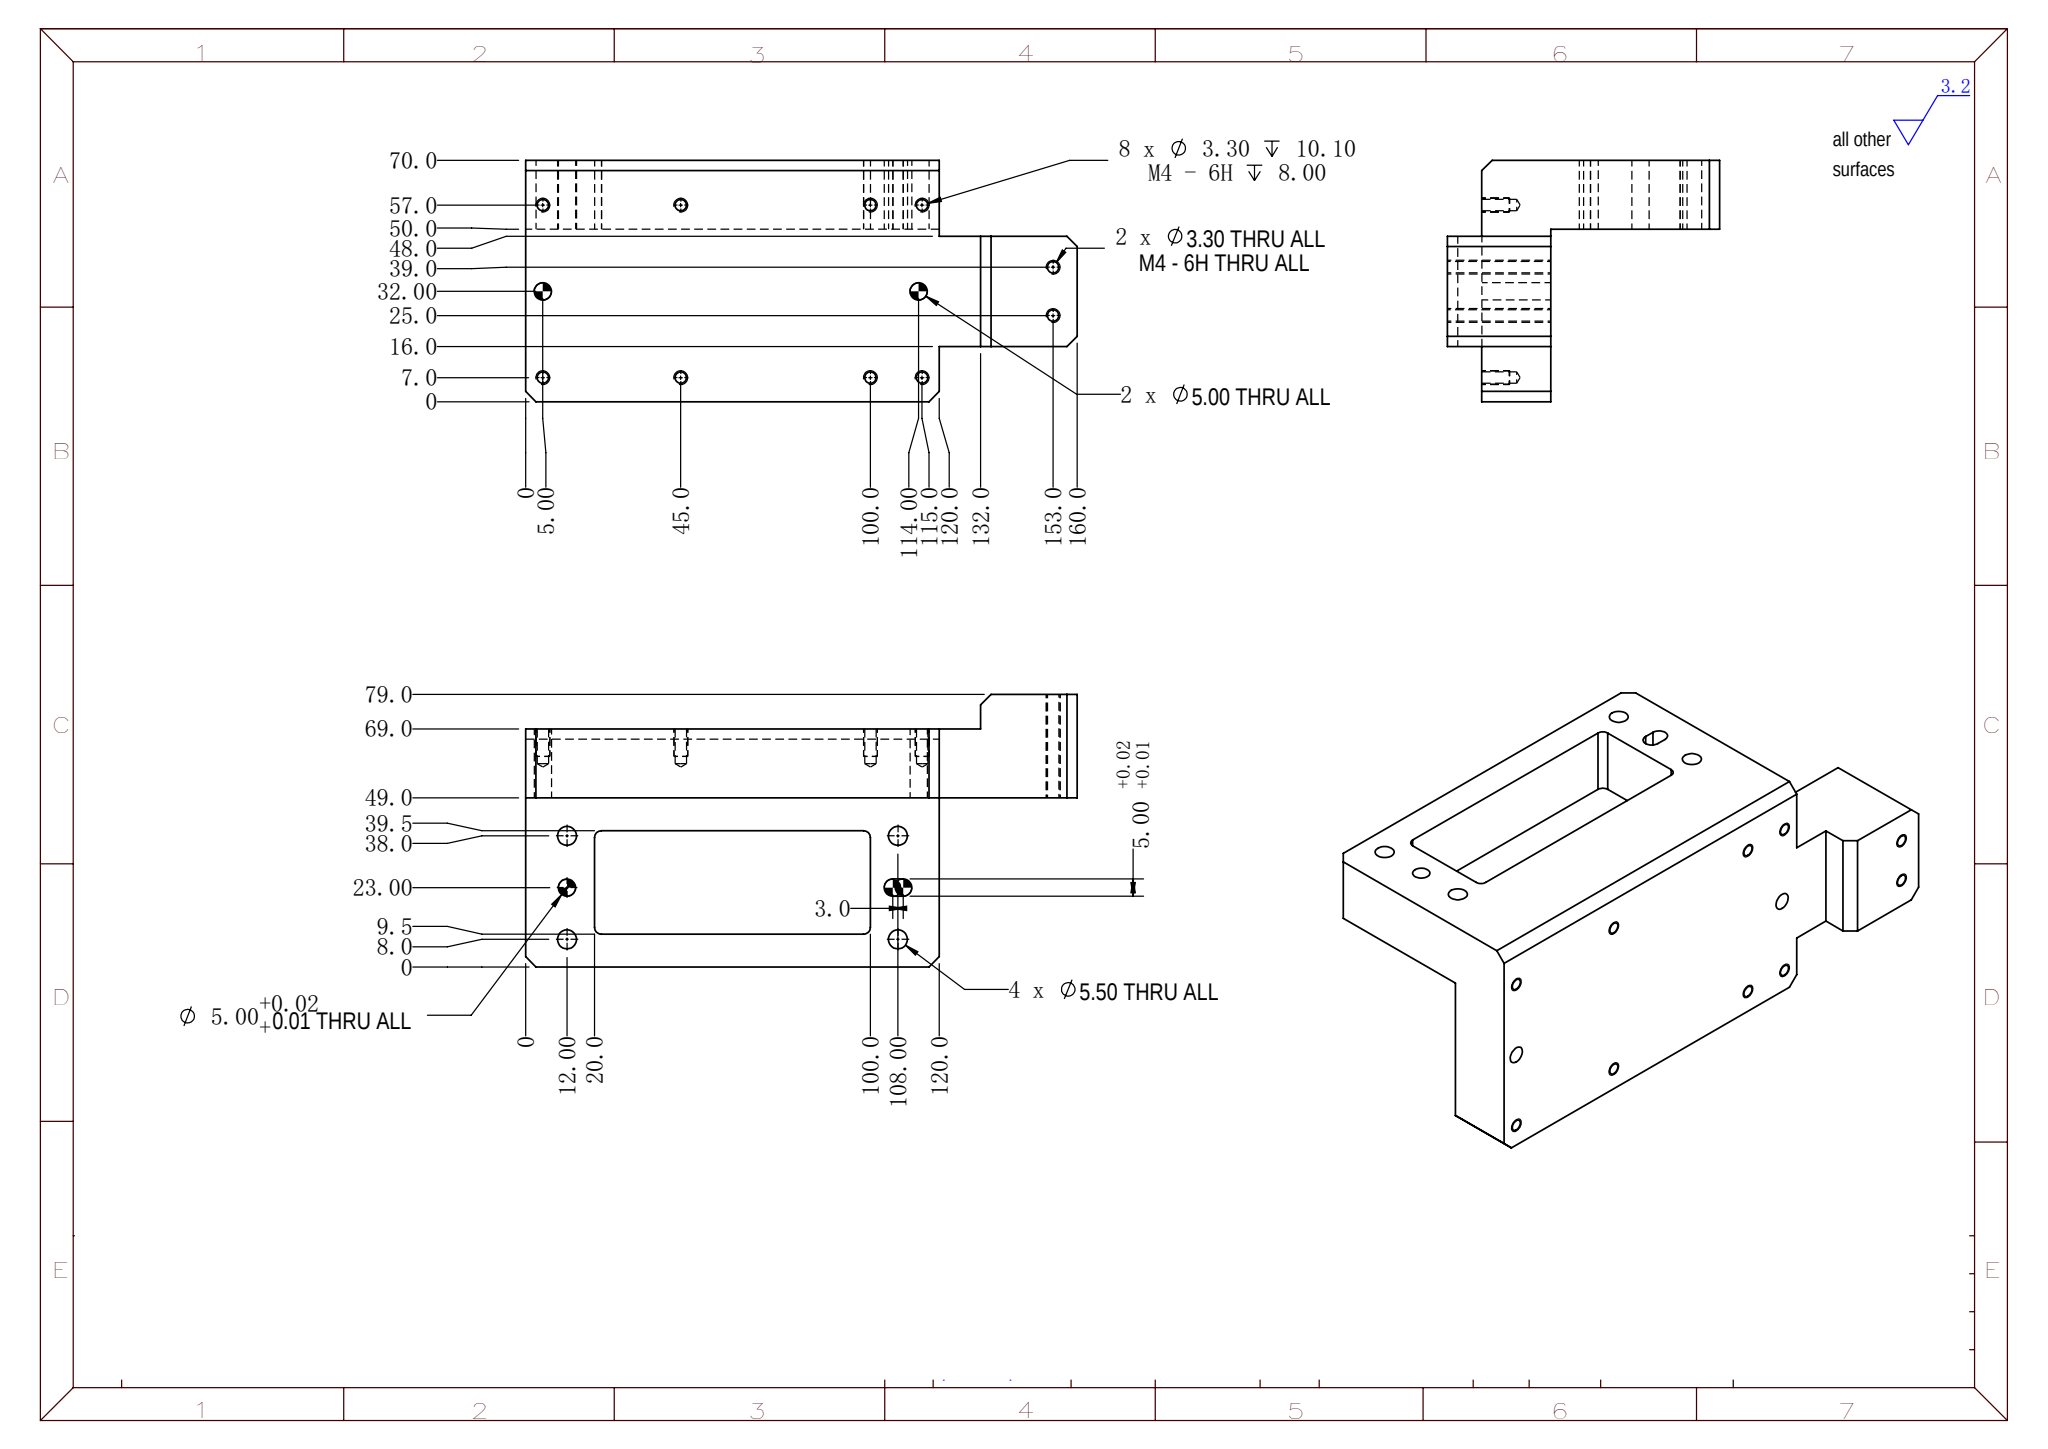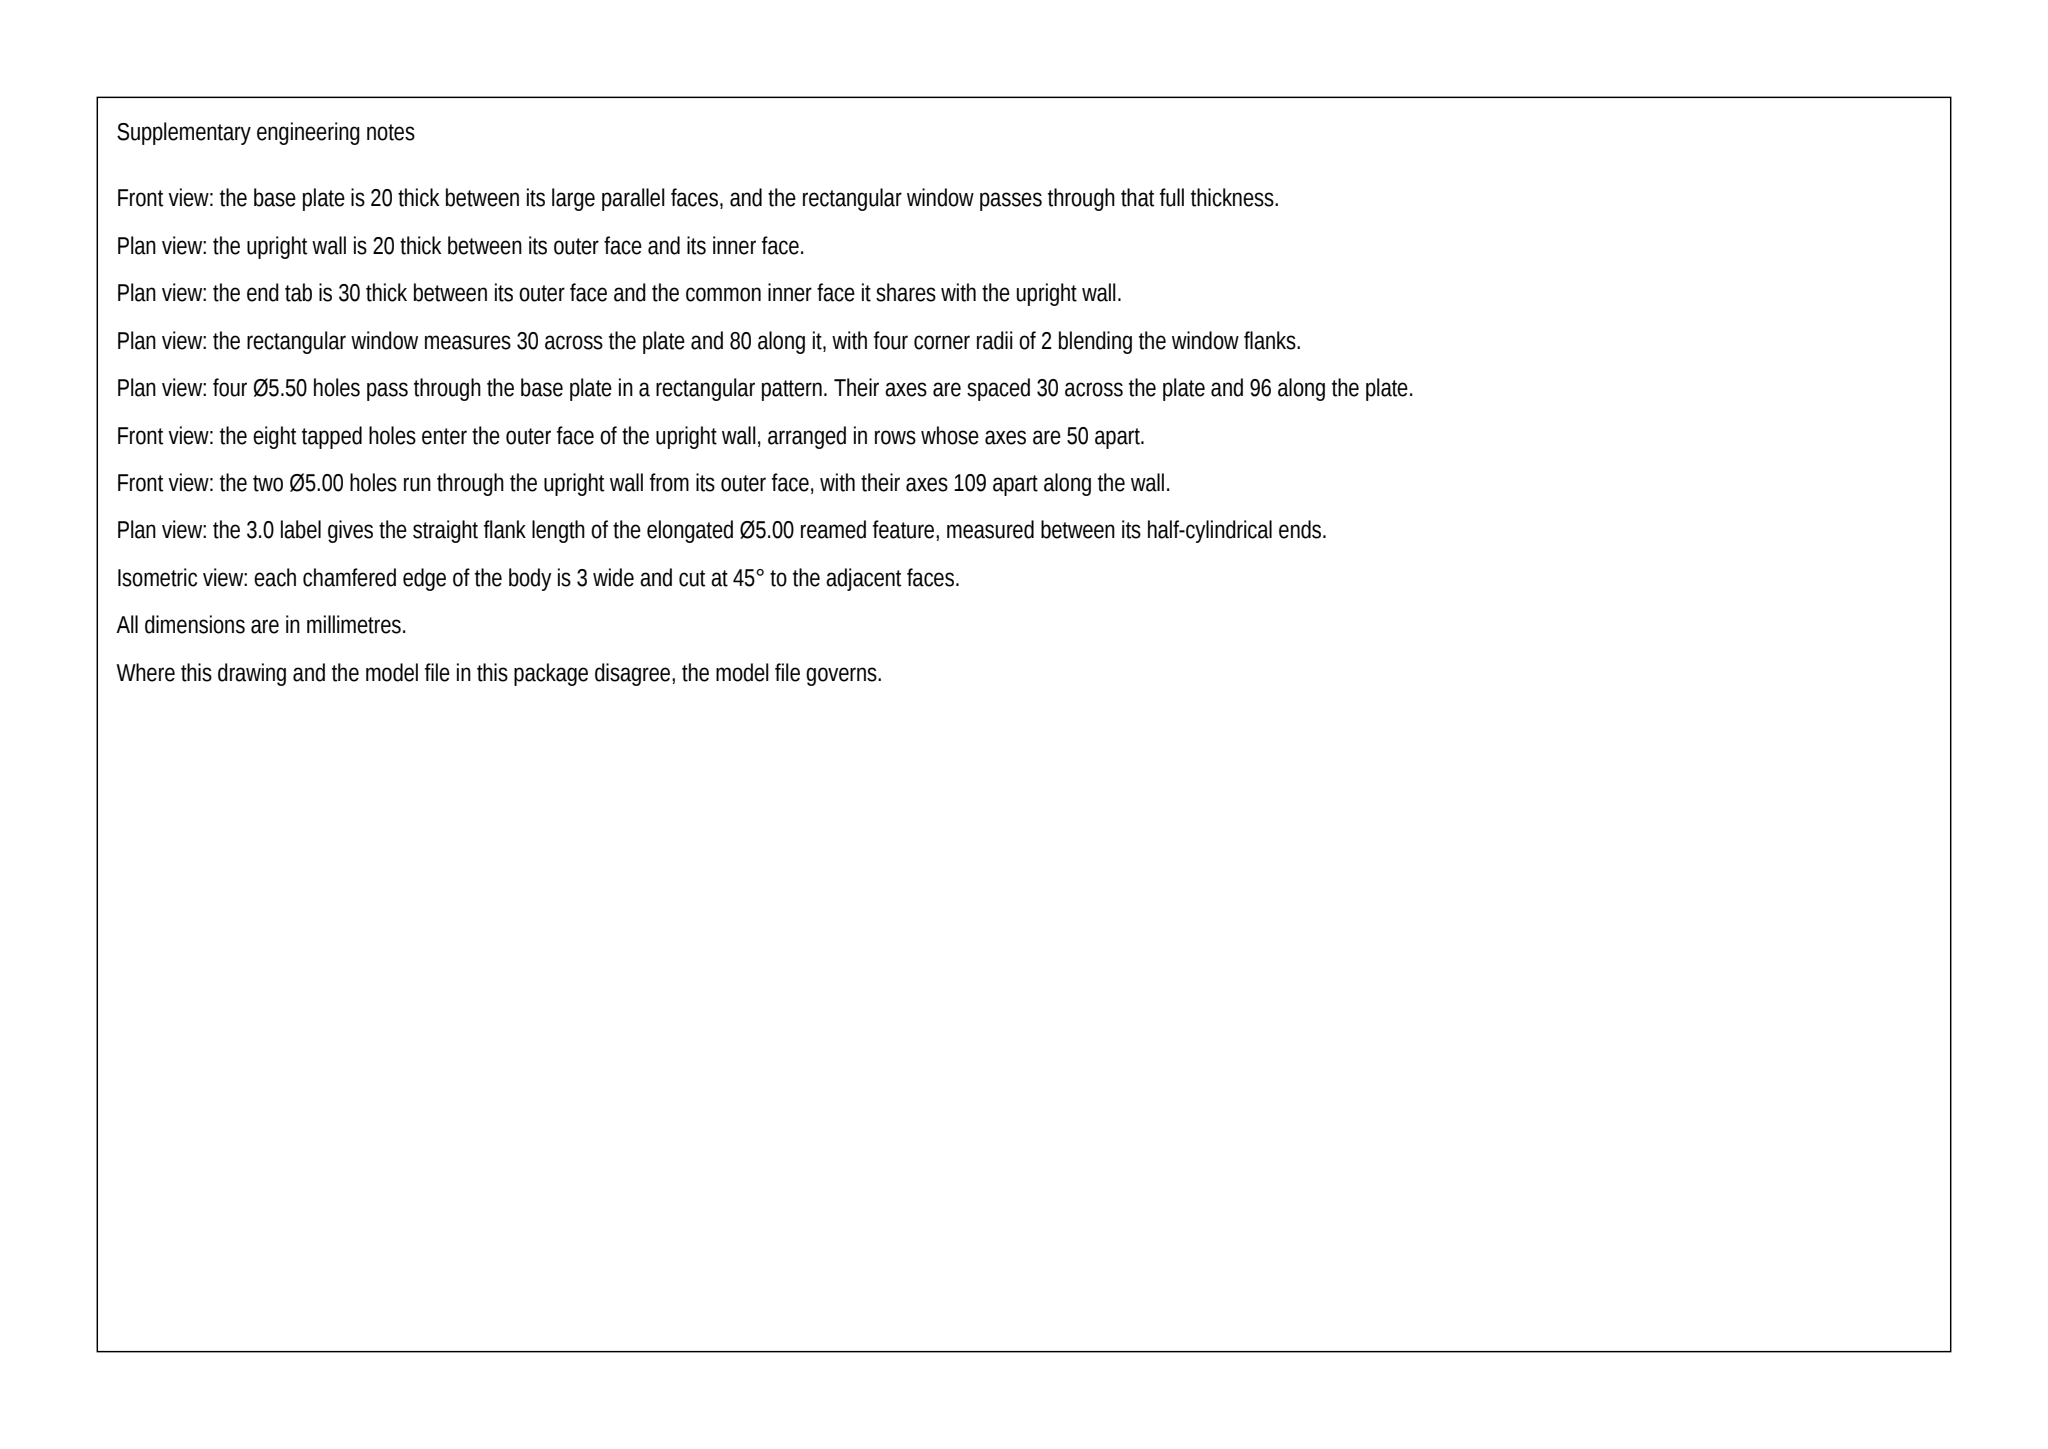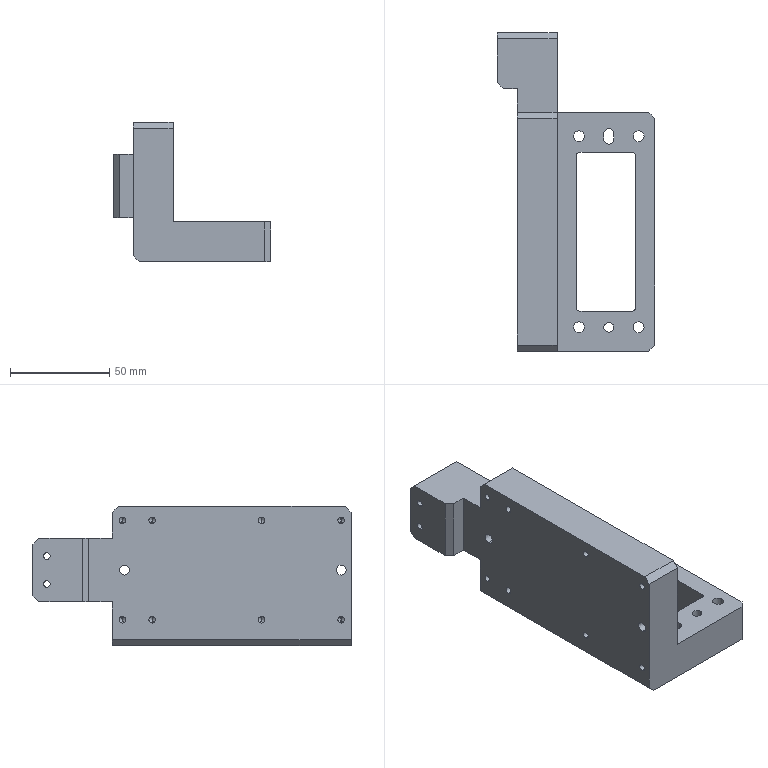Part | SolidWorks | mm | 1 solid | 84 faces | box 79 x 160 x 70 mm | volume 265916 mm3 | cylinder 40 | plane 28 | cone 16 | commonest cylinder face diameters 3.3 x20 5 x8 5.5 x8 4 x4
Drawing notes:
POCKET 30 X 80: CORNER R2 (4X), FULL DEPTH | from the solid: Ø4 z-axis cyls at (41.5,22),(41.5,98),(67.5,22),(67.5,98) = R2 corners of pocket bounded by x39.5-69.5, y20-100
2X Ø5.00 HOLES ON X AXIS (AT Y5.00 AND Y114.00): 20.0 DEEP, BLIND | from the solid: cylinders [5.0,"x",[null,5.0,38.0],20.0] and [5.0,"x",[null,114.0,38.0],20.0] - length 20.0, not through 79.0 bbox width
5.00 (+0.02/+0.01) WIDE STEP ON END FLANGE: FACES LOCATED AT X53.5 AND X58.5 FROM DATUM FACE X0 (BBOX MIN) | from the solid: axis_planes ["x",53.5,1] and ["x",58.5,1]; bbox_xyz x=79.0 measured from min corner
build123d program:
from build123d import *

# Parameters (mm, degrees)
SKETCH1_W                  = 80
SKETCH1_H                  = 160
BOSS_EXTRUDE1_DEPTH        = 35
SKETCH2_W                  = 70
SKETCH2_H                  = 120
CUT_EXTRUDE1_DEPTH         = 11
SKETCH4_W                  = 49
SKETCH4_H                  = 50
CUT_EXTRUDE2_DEPTH         = 169.597
SKETCH6_W                  = 80
SKETCH6_H                  = 40
CUT_EXTRUDE4_DEPTH         = 22
SKETCH7_W                  = 16
SKETCH7_H                  = 40
CUT_EXTRUDE5_DEPTH         = 119.427
M4_TAPPED_HOLE1_D          = 3.3
M4_TAPPED_HOLE2_D          = 3.3
M4_TAPPED_HOLE2_DEPTH      = 10.1
M4_TAPPED_HOLE2_TIP        = 0.9914
SIZE_MM_DOWEL_PIN_HOLE1_D  = 5
F_5_5_5_5_DIAMETER_HOLE1_D = 5.5
CUT_EXTRUDE6_DEPTH         = 105.48
CUT_EXTRUDE7_DEPTH         = 103.47
F_5_0_5_DIAMETER_HOLE1_D   = 5
CUT_EXTRUDE8_DEPTH         = 103.47
CHAMFER1_SIZE              = 3
SKETCH26_W                 = 11
SKETCH26_H                 = 12
CUT_EXTRUDE9_DEPTH         = 114.578
SKETCH27_W                 = 1
SKETCH27_H                 = 28
CUT_EXTRUDE10_DEPTH        = 105.48
CHAMFER3_SIZE              = 3


with BuildPart() as part:
    # Sketch1 → Boss-Extrude1 (new, symmetric)
    with BuildSketch(Plane.XY):
        Rectangle(SKETCH1_W, SKETCH1_H)
    extrude(amount=BOSS_EXTRUDE1_DEPTH, both=True)

    # Sketch2 → Cut-Extrude1 (cut)
    with BuildSketch(Plane.ZY.offset(40)):
        with Locations((0, -20)):
            Rectangle(SKETCH2_W, SKETCH2_H)
    extrude(amount=-CUT_EXTRUDE1_DEPTH, mode=Mode.SUBTRACT)

    # Sketch4 → Cut-Extrude2 (cut, through all)
    with BuildSketch(Plane.XZ.offset(80)):
        with Locations((15.5, 10)):
            Rectangle(SKETCH4_W, SKETCH4_H)
    extrude(amount=-CUT_EXTRUDE2_DEPTH, mode=Mode.SUBTRACT)

    # Sketch6 → Cut-Extrude4 (cut)
    with BuildSketch(Plane(origin=(0, 0, -35), x_dir=(-1, 0, 0), z_dir=(0, 0, -1))):
        with Locations((0, 60)):
            Rectangle(SKETCH6_W, SKETCH6_H)
    extrude(amount=-CUT_EXTRUDE4_DEPTH, mode=Mode.SUBTRACT)

    # Sketch7 → Cut-Extrude5 (cut, through all)
    with BuildSketch(Plane.ZY.offset(40)):
        with Locations((27, 60)):
            Rectangle(SKETCH7_W, SKETCH7_H)
    extrude(amount=-CUT_EXTRUDE5_DEPTH, mode=Mode.SUBTRACT)

    # M4 Tapped Hole1 (through all)
    with Locations(Plane.ZY.offset(40)):
        with Locations((10, 73), (-4, 73)):
            Hole(M4_TAPPED_HOLE1_D / 2)

    # M4 Tapped Hole2
    with Locations(Plane.ZY.offset(29)):
        with Locations((-22, -75), (-22, -35), (-22, 20), (-22, 35), (28, 35), (28, 20), (28, -35), (28, -75)):
            Hole(M4_TAPPED_HOLE2_D / 2, depth=M4_TAPPED_HOLE2_DEPTH)
            with Locations((0, 0, -(M4_TAPPED_HOLE2_DEPTH + M4_TAPPED_HOLE2_TIP / 2))):  # 118° drill point
                Cone(0, M4_TAPPED_HOLE2_D / 2, M4_TAPPED_HOLE2_TIP, mode=Mode.SUBTRACT)

    # Size mm Dowel Pin Hole1 (through all)
    with Locations(Plane.ZY.offset(29)):
        with Locations((3, -75), (3, 34)):
            Hole(SIZE_MM_DOWEL_PIN_HOLE1_D / 2)

    # 5.5 _5.5_ Diameter Hole1 (through all)
    with Locations(Plane.XY.offset(-15)):
        with Locations((2, 28), (32, 28), (2, -68), (32, -68)):
            Hole(F_5_5_5_5_DIAMETER_HOLE1_D / 2)

    # Sketch21 → Cut-Extrude6 (cut, through all)
    with BuildSketch(Plane.XY.offset(19)):
        Polygon((-29, 40), (-40, 51), (-40, 40), align=None)
    extrude(amount=-CUT_EXTRUDE6_DEPTH, mode=Mode.SUBTRACT)

    # Sketch22 → Cut-Extrude7 (cut, through all)
    with BuildSketch(Plane.XY.offset(-15)):
        with BuildLine():
            Line((28.5, -60), (2.5, -60))
            ThreePointArc((2.5, -60), (1.086, -59.414), (0.5, -58))
            Line((0.5, -58), (0.5, 18))
            ThreePointArc((0.5, 18), (1.086, 19.414), (2.5, 20))
            Line((2.5, 20), (28.5, 20))
            ThreePointArc((28.5, 20), (29.914, 19.414), (30.5, 18))
            Line((30.5, 18), (30.5, -58))
            ThreePointArc((30.5, -58), (29.914, -59.414), (28.5, -60))
        make_face()
    extrude(amount=-CUT_EXTRUDE7_DEPTH, mode=Mode.SUBTRACT)

    # 5.0 _5_ Diameter Hole1 (through all)
    with Locations(Plane.XY.offset(-15)):
        with Locations((17, -68), (17, 28)):
            Hole(F_5_0_5_DIAMETER_HOLE1_D / 2)

    # Sketch25 → Cut-Extrude8 (cut, through all)
    with BuildSketch(Plane.XY.offset(-15)):
        with BuildLine():
            Line((14.5, 26.5), (14.5, 29.5))
            ThreePointArc((14.5, 29.5), (17, 32), (19.5, 29.5))
            Line((19.5, 29.5), (19.5, 26.5))
            ThreePointArc((19.5, 26.5), (17, 24), (14.5, 26.5))
        make_face()
    extrude(amount=-CUT_EXTRUDE8_DEPTH, mode=Mode.SUBTRACT)

    # Chamfer1
    chamfer1_edges = [part.edges().sort_by_distance(p)[0] for p in [
        (-19, -80, 35),
        (-29, -20, -35),
        (40, -80, -25),
        (40, 40, -25),
        (-24.5, 80, -13),
        (-19, 40, 35),
        (-24.5, 80, 19),
    ]]
    chamfer(chamfer1_edges, length=CHAMFER1_SIZE)

    # Sketch26 → Cut-Extrude9 (cut, through all)
    with BuildSketch(Plane.XY.offset(35)):
        with Locations((-34.5, 46)):
            Rectangle(SKETCH26_W, SKETCH26_H)
    extrude(amount=-CUT_EXTRUDE9_DEPTH, mode=Mode.SUBTRACT)

    # Sketch27 → Cut-Extrude10 (cut, through all)
    with BuildSketch(Plane.XY.offset(19)):
        with Locations((-39.5, 66)):
            Rectangle(SKETCH27_W, SKETCH27_H)
    extrude(amount=-CUT_EXTRUDE10_DEPTH, mode=Mode.SUBTRACT)

    # Chamfer3
    chamfer3_edges = [part.edges().sort_by_distance(p)[0] for p in [
        (-39, 52, 3),
    ]]
    chamfer(chamfer3_edges, length=CHAMFER3_SIZE)


solid = part.part